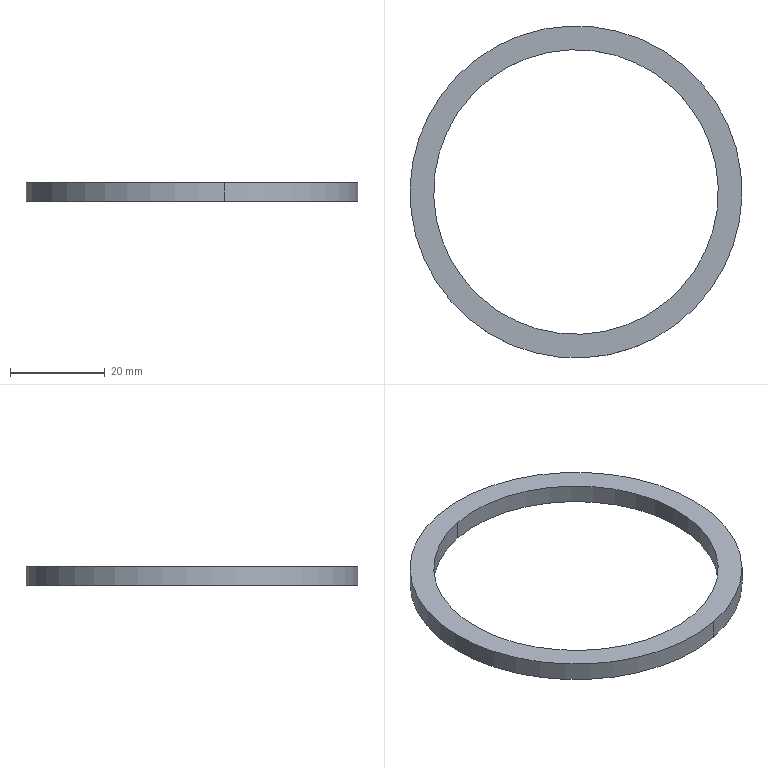Component | SolidWorks | BearingRetainingRing-1 | 1 solid | 6 faces | box 70 x 70 x 4 mm | volume 4084 mm3 | cylinder 4 | plane 2 | commonest cylinder face diameters 60 x2 70 x2
build123d program:
from build123d import *

# Parameters (mm, degrees)
SKETCH1_R           = 35
SKETCH1_R_2         = 30
BOSS_EXTRUDE1_DEPTH = 4


with BuildPart() as part:
    # Sketch1 → Boss-Extrude1 (new body)
    with BuildSketch(Plane(origin=(0, 0, 0), x_dir=(1, 0, 0), z_dir=(0, 1, 0))):
        with Locations(Location((0, 0, 0), (0, 0, 270))):
            Circle(SKETCH1_R)
        with Locations(Location((0, 0, 0), (0, 0, 270))):
            Circle(SKETCH1_R_2, mode=Mode.SUBTRACT)
    extrude(amount=BOSS_EXTRUDE1_DEPTH)


solid = part.part

# Placed as in the assembly
solid = solid.moved(Location((-85, 178, 115), (90, 0, 0)))
STEP:
#1=COLOUR_RGB('',0.7922,0.8196,0.9333);
#2=FILL_AREA_STYLE_COLOUR('',#1);
#3=FILL_AREA_STYLE('',(#2));
#4=SURFACE_STYLE_FILL_AREA(#3);
#5=SURFACE_SIDE_STYLE('',(#4));
#6=SURFACE_STYLE_USAGE(.BOTH.,#5);
#7=PRESENTATION_STYLE_ASSIGNMENT((#6));
#8=CARTESIAN_POINT('',(-3.118,5.849,4.528));
#9=VERTEX_POINT('',#8);
#10=CARTESIAN_POINT('',(-3.574,8.167,4.528));
#11=VERTEX_POINT('',#10);
#12=CARTESIAN_POINT('',(-3.346,7.008,4.528));
#13=DIRECTION('',(-0.,0.,-1.));
#14=DIRECTION('',(-0.193,0.9812,0.));
#15=AXIS2_PLACEMENT_3D('',#12,#13,#14);
#16=CIRCLE('',#15,1.181);
#17=EDGE_CURVE('',#9,#11,#16,.T.);
#18=ORIENTED_EDGE('',*,*,#17,.T.);
#19=CARTESIAN_POINT('',(-3.574,8.167,4.685));
#20=VERTEX_POINT('',#19);
#21=CARTESIAN_POINT('',(-3.574,8.167,4.528));
#22=DIRECTION('',(0.,-0.,1.));
#23=VECTOR('',#22,39.37);
#24=LINE('',#21,#23);
#25=EDGE_CURVE('',#11,#20,#24,.T.);
#26=ORIENTED_EDGE('',*,*,#25,.T.);
#27=CARTESIAN_POINT('',(-3.118,5.849,4.685));
#28=VERTEX_POINT('',#27);
#29=CARTESIAN_POINT('',(-3.346,7.008,4.685));
#30=DIRECTION('',(-0.,0.,-1.));
#31=DIRECTION('',(-0.193,0.9812,0.));
#32=AXIS2_PLACEMENT_3D('',#29,#30,#31);
#33=CIRCLE('',#32,1.181);
#34=EDGE_CURVE('',#28,#20,#33,.T.);
#35=ORIENTED_EDGE('',*,*,#34,.F.);
#36=CARTESIAN_POINT('',(-3.118,5.849,4.528));
#37=DIRECTION('',(0.,-0.,1.));
#38=VECTOR('',#37,39.37);
#39=LINE('',#36,#38);
#40=EDGE_CURVE('',#9,#28,#39,.T.);
#41=ORIENTED_EDGE('',*,*,#40,.F.);
#42=EDGE_LOOP('',(#18,#26,#35,#41));
#43=FACE_OUTER_BOUND('',#42,.T.);
#44=CARTESIAN_POINT('',(-3.346,7.008,4.528));
#45=DIRECTION('',(0.,-0.,1.));
#46=DIRECTION('',(0.193,-0.9812,-0.));
#47=AXIS2_PLACEMENT_3D('',#44,#45,#46);
#48=CYLINDRICAL_SURFACE('',#47,1.181);
#49=ADVANCED_FACE('',(#43),#48,.F.);
#50=CARTESIAN_POINT('',(-3.612,8.36,4.528));
#51=VERTEX_POINT('',#50);
#52=CARTESIAN_POINT('',(-3.08,5.656,4.528));
#53=VERTEX_POINT('',#52);
#54=CARTESIAN_POINT('',(-3.346,7.008,4.528));
#55=DIRECTION('',(-0.,0.,-1.));
#56=DIRECTION('',(-0.193,0.9812,0.));
#57=AXIS2_PLACEMENT_3D('',#54,#55,#56);
#58=CIRCLE('',#57,1.378);
#59=EDGE_CURVE('',#51,#53,#58,.T.);
#60=ORIENTED_EDGE('',*,*,#59,.F.);
#61=CARTESIAN_POINT('',(-3.612,8.36,4.685));
#62=VERTEX_POINT('',#61);
#63=CARTESIAN_POINT('',(-3.612,8.36,4.528));
#64=DIRECTION('',(0.,-0.,1.));
#65=VECTOR('',#64,39.37);
#66=LINE('',#63,#65);
#67=EDGE_CURVE('',#51,#62,#66,.T.);
#68=ORIENTED_EDGE('',*,*,#67,.T.);
#69=CARTESIAN_POINT('',(-3.08,5.656,4.685));
#70=VERTEX_POINT('',#69);
#71=CARTESIAN_POINT('',(-3.346,7.008,4.685));
#72=DIRECTION('',(-0.,0.,-1.));
#73=DIRECTION('',(-0.193,0.9812,0.));
#74=AXIS2_PLACEMENT_3D('',#71,#72,#73);
#75=CIRCLE('',#74,1.378);
#76=EDGE_CURVE('',#62,#70,#75,.T.);
#77=ORIENTED_EDGE('',*,*,#76,.T.);
#78=CARTESIAN_POINT('',(-3.08,5.656,4.528));
#79=DIRECTION('',(0.,-0.,1.));
#80=VECTOR('',#79,39.37);
#81=LINE('',#78,#80);
#82=EDGE_CURVE('',#53,#70,#81,.T.);
#83=ORIENTED_EDGE('',*,*,#82,.F.);
#84=EDGE_LOOP('',(#60,#68,#77,#83));
#85=FACE_OUTER_BOUND('',#84,.T.);
#86=CARTESIAN_POINT('',(-3.346,7.008,4.528));
#87=DIRECTION('',(0.,-0.,1.));
#88=DIRECTION('',(0.193,-0.9812,-0.));
#89=AXIS2_PLACEMENT_3D('',#86,#87,#88);
#90=CYLINDRICAL_SURFACE('',#89,1.378);
#91=ADVANCED_FACE('',(#85),#90,.T.);
#92=CARTESIAN_POINT('',(-3.346,7.008,4.528));
#93=DIRECTION('',(-0.,0.,-1.));
#94=DIRECTION('',(-0.193,0.9812,0.));
#95=AXIS2_PLACEMENT_3D('',#92,#93,#94);
#96=CIRCLE('',#95,1.378);
#97=EDGE_CURVE('',#53,#51,#96,.T.);
#98=ORIENTED_EDGE('',*,*,#97,.T.);
#99=ORIENTED_EDGE('',*,*,#59,.T.);
#100=EDGE_LOOP('',(#98,#99));
#101=FACE_OUTER_BOUND('',#100,.T.);
#102=ORIENTED_EDGE('',*,*,#17,.F.);
#103=CARTESIAN_POINT('',(-3.346,7.008,4.528));
#104=DIRECTION('',(-0.,0.,-1.));
#105=DIRECTION('',(-0.193,0.9812,0.));
#106=AXIS2_PLACEMENT_3D('',#103,#104,#105);
#107=CIRCLE('',#106,1.181);
#108=EDGE_CURVE('',#11,#9,#107,.T.);
#109=ORIENTED_EDGE('',*,*,#108,.F.);
#110=EDGE_LOOP('',(#102,#109));
#111=FACE_BOUND('',#110,.T.);
#112=CARTESIAN_POINT('',(-3.346,7.008,4.528));
#113=DIRECTION('',(-0.,0.,-1.));
#114=DIRECTION('',(-0.193,0.9812,0.));
#115=AXIS2_PLACEMENT_3D('',#112,#113,#114);
#116=PLANE('',#115);
#117=ADVANCED_FACE('',(#101,#111),#116,.T.);
#118=CARTESIAN_POINT('',(-3.346,7.008,4.685));
#119=DIRECTION('',(-0.,0.,-1.));
#120=DIRECTION('',(-0.193,0.9812,0.));
#121=AXIS2_PLACEMENT_3D('',#118,#119,#120);
#122=CIRCLE('',#121,1.378);
#123=EDGE_CURVE('',#70,#62,#122,.T.);
#124=ORIENTED_EDGE('',*,*,#123,.F.);
#125=ORIENTED_EDGE('',*,*,#76,.F.);
#126=EDGE_LOOP('',(#124,#125));
#127=FACE_OUTER_BOUND('',#126,.T.);
#128=ORIENTED_EDGE('',*,*,#34,.T.);
#129=CARTESIAN_POINT('',(-3.346,7.008,4.685));
#130=DIRECTION('',(-0.,0.,-1.));
#131=DIRECTION('',(-0.193,0.9812,0.));
#132=AXIS2_PLACEMENT_3D('',#129,#130,#131);
#133=CIRCLE('',#132,1.181);
#134=EDGE_CURVE('',#20,#28,#133,.T.);
#135=ORIENTED_EDGE('',*,*,#134,.T.);
#136=EDGE_LOOP('',(#128,#135));
#137=FACE_BOUND('',#136,.T.);
#138=CARTESIAN_POINT('',(-3.346,7.008,4.685));
#139=DIRECTION('',(-0.,0.,-1.));
#140=DIRECTION('',(-0.193,0.9812,0.));
#141=AXIS2_PLACEMENT_3D('',#138,#139,#140);
#142=PLANE('',#141);
#143=ADVANCED_FACE('',(#127,#137),#142,.F.);
#144=ORIENTED_EDGE('',*,*,#67,.F.);
#145=ORIENTED_EDGE('',*,*,#97,.F.);
#146=ORIENTED_EDGE('',*,*,#82,.T.);
#147=ORIENTED_EDGE('',*,*,#123,.T.);
#148=EDGE_LOOP('',(#144,#145,#146,#147));
#149=FACE_OUTER_BOUND('',#148,.T.);
#150=CARTESIAN_POINT('',(-3.346,7.008,4.528));
#151=DIRECTION('',(0.,-0.,1.));
#152=DIRECTION('',(0.193,-0.9812,-0.));
#153=AXIS2_PLACEMENT_3D('',#150,#151,#152);
#154=CYLINDRICAL_SURFACE('',#153,1.378);
#155=ADVANCED_FACE('',(#149),#154,.T.);
#156=ORIENTED_EDGE('',*,*,#25,.F.);
#157=ORIENTED_EDGE('',*,*,#108,.T.);
#158=ORIENTED_EDGE('',*,*,#40,.T.);
#159=ORIENTED_EDGE('',*,*,#134,.F.);
#160=EDGE_LOOP('',(#156,#157,#158,#159));
#161=FACE_OUTER_BOUND('',#160,.T.);
#162=CARTESIAN_POINT('',(-3.346,7.008,4.528));
#163=DIRECTION('',(0.,-0.,1.));
#164=DIRECTION('',(0.193,-0.9812,-0.));
#165=AXIS2_PLACEMENT_3D('',#162,#163,#164);
#166=CYLINDRICAL_SURFACE('',#165,1.181);
#167=ADVANCED_FACE('',(#161),#166,.F.);
#168=CLOSED_SHELL('',(#49,#91,#117,#143,#155,#167));
#169=MANIFOLD_SOLID_BREP('',#168);
#170=STYLED_ITEM('',(#7),#169);
#171=PRESENTATION_LAYER_ASSIGNMENT('','',(#170));
#172=CARTESIAN_POINT('',(0.,0.,0.));
#173=DIRECTION('',(0.,0.,1.));
#174=DIRECTION('',(1.,0.,0.));
#175=AXIS2_PLACEMENT_3D('',#172,#173,#174);
#176=(LENGTH_UNIT()NAMED_UNIT(*)SI_UNIT($,.METRE.));
#177=LENGTH_MEASURE_WITH_UNIT(LENGTH_MEASURE(0.0254),#176);
#178=DIMENSIONAL_EXPONENTS(1.,0.,0.,0.,0.,0.,0.);
#179=(CONVERSION_BASED_UNIT('',#177)LENGTH_UNIT()NAMED_UNIT(#178));
#180=UNCERTAINTY_MEASURE_WITH_UNIT(LENGTH_MEASURE(0.00001),#179,'','');
#181=(NAMED_UNIT(*)PLANE_ANGLE_UNIT()SI_UNIT($,.RADIAN.));
#182=(NAMED_UNIT(*)SI_UNIT($,.STERADIAN.)SOLID_ANGLE_UNIT());
#183=(GEOMETRIC_REPRESENTATION_CONTEXT(3)GLOBAL_UNCERTAINTY_ASSIGNED_CONTEXT((#180))GLOBAL_UNIT_ASSIGNED_CONTEXT((#179,#181,#182))REPRESENTATION_CONTEXT('',''));
#184=ADVANCED_BREP_SHAPE_REPRESENTATION('',(#169,#175),#183);
#185=(LENGTH_UNIT()NAMED_UNIT(*)SI_UNIT($,.METRE.));
#186=LENGTH_MEASURE_WITH_UNIT(LENGTH_MEASURE(0.0254),#185);
#187=DIMENSIONAL_EXPONENTS(1.,0.,0.,0.,0.,0.,0.);
#188=(CONVERSION_BASED_UNIT('',#186)LENGTH_UNIT()NAMED_UNIT(#187));
#189=UNCERTAINTY_MEASURE_WITH_UNIT(LENGTH_MEASURE(0.00001),#188,'','');
#190=(NAMED_UNIT(*)PLANE_ANGLE_UNIT()SI_UNIT($,.RADIAN.));
#191=(NAMED_UNIT(*)SI_UNIT($,.STERADIAN.)SOLID_ANGLE_UNIT());
#192=(GEOMETRIC_REPRESENTATION_CONTEXT(3)GLOBAL_UNCERTAINTY_ASSIGNED_CONTEXT((#189))GLOBAL_UNIT_ASSIGNED_CONTEXT((#188,#190,#191))REPRESENTATION_CONTEXT('',''));
#193=MECHANICAL_DESIGN_GEOMETRIC_PRESENTATION_REPRESENTATION('',(#170),#192);